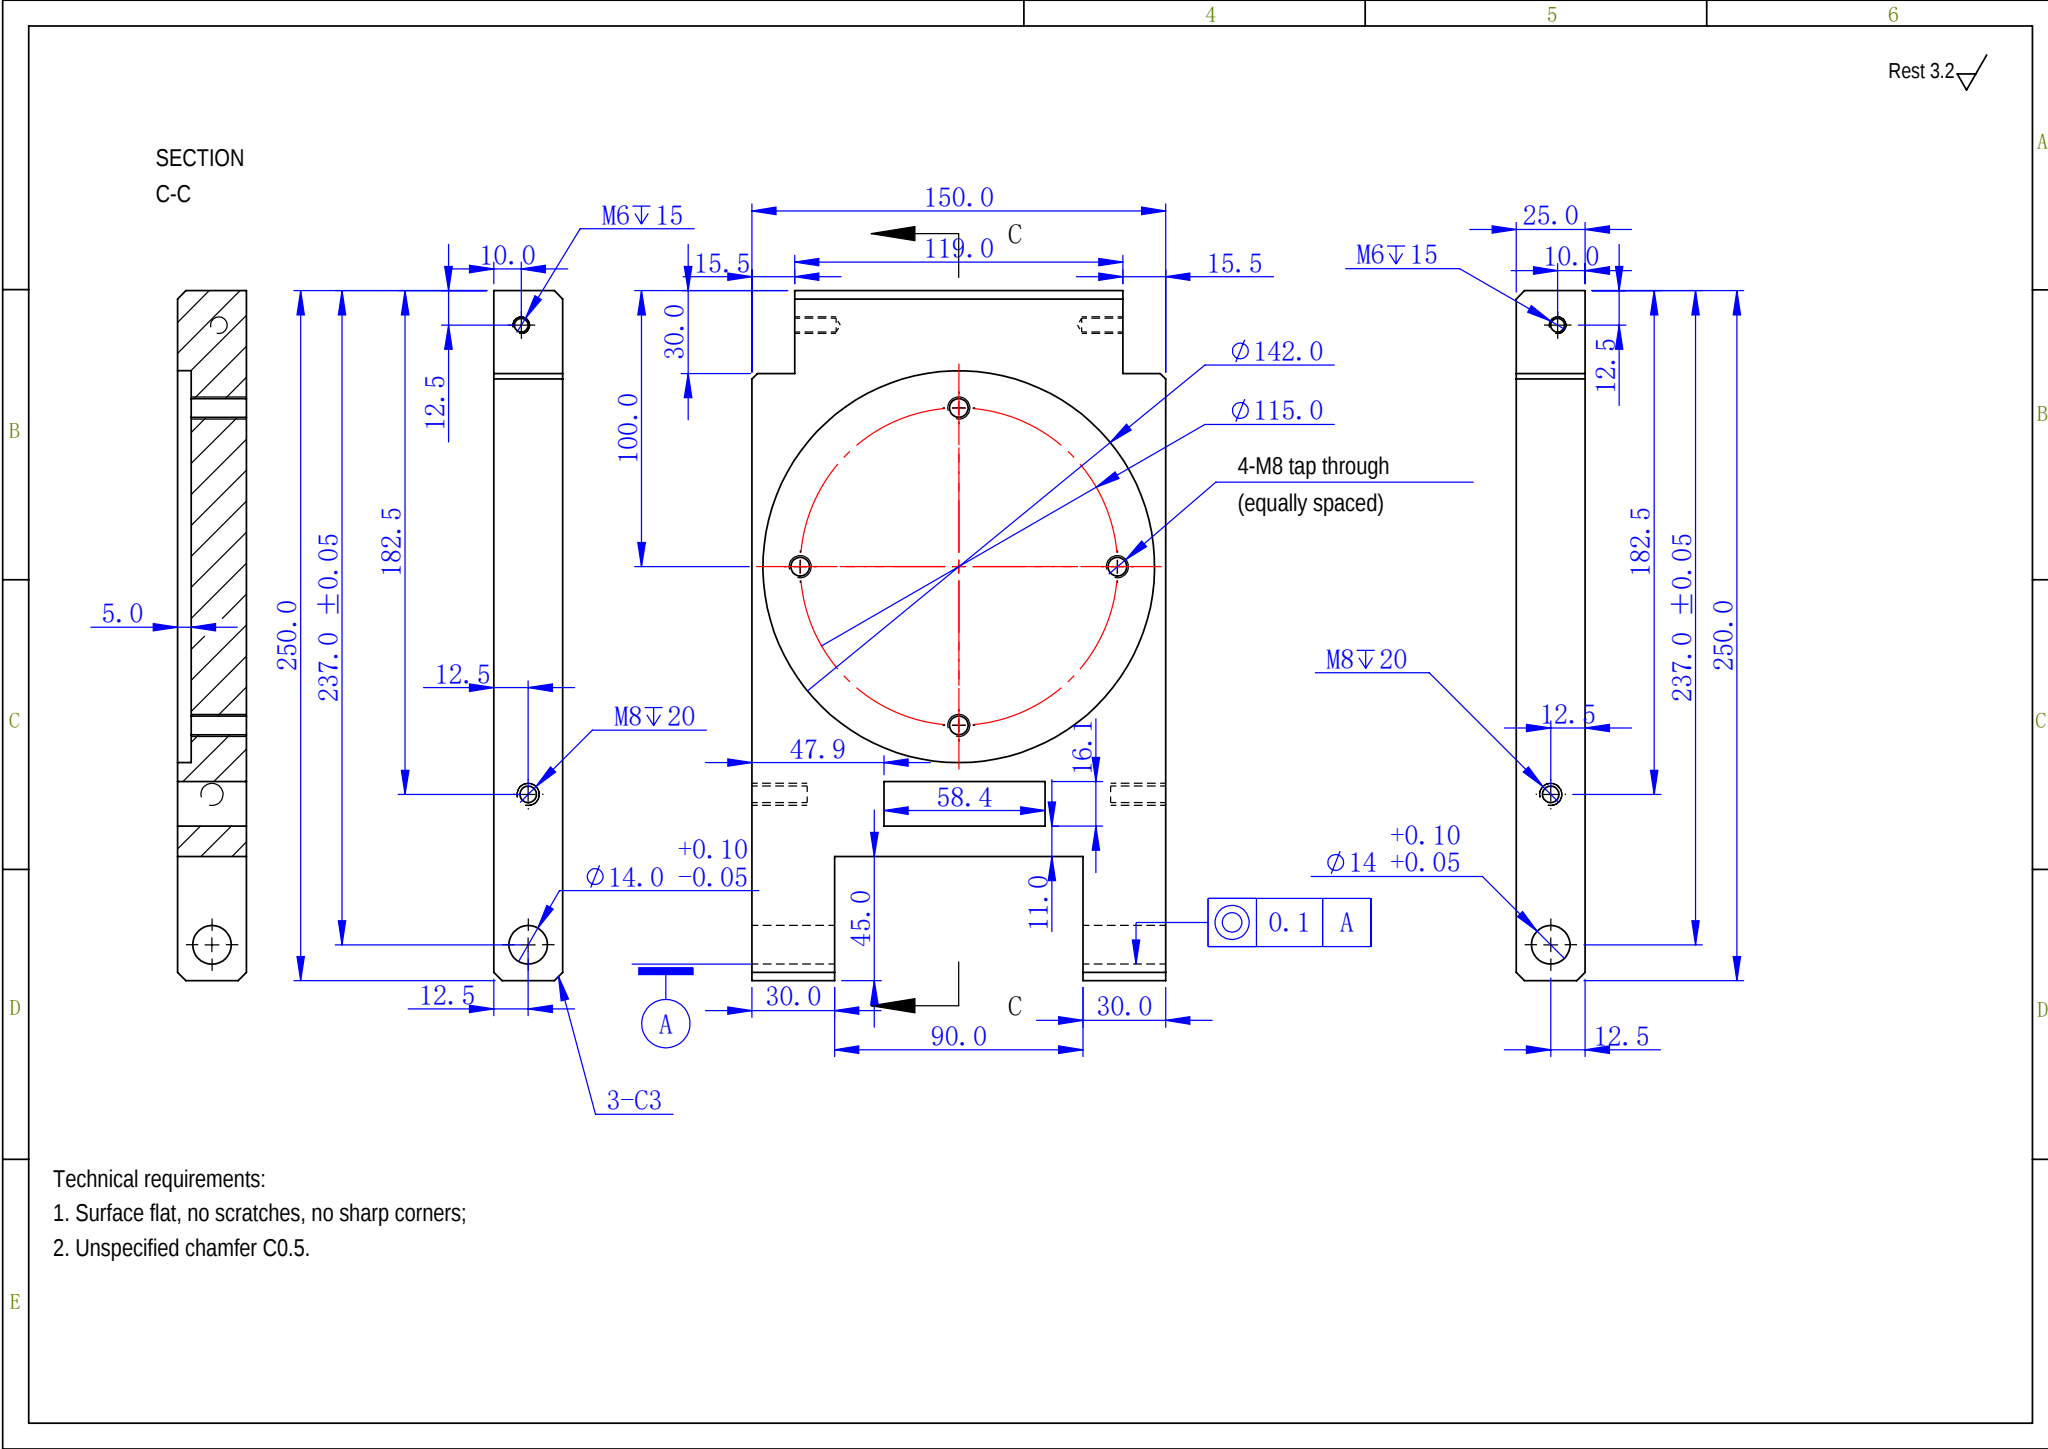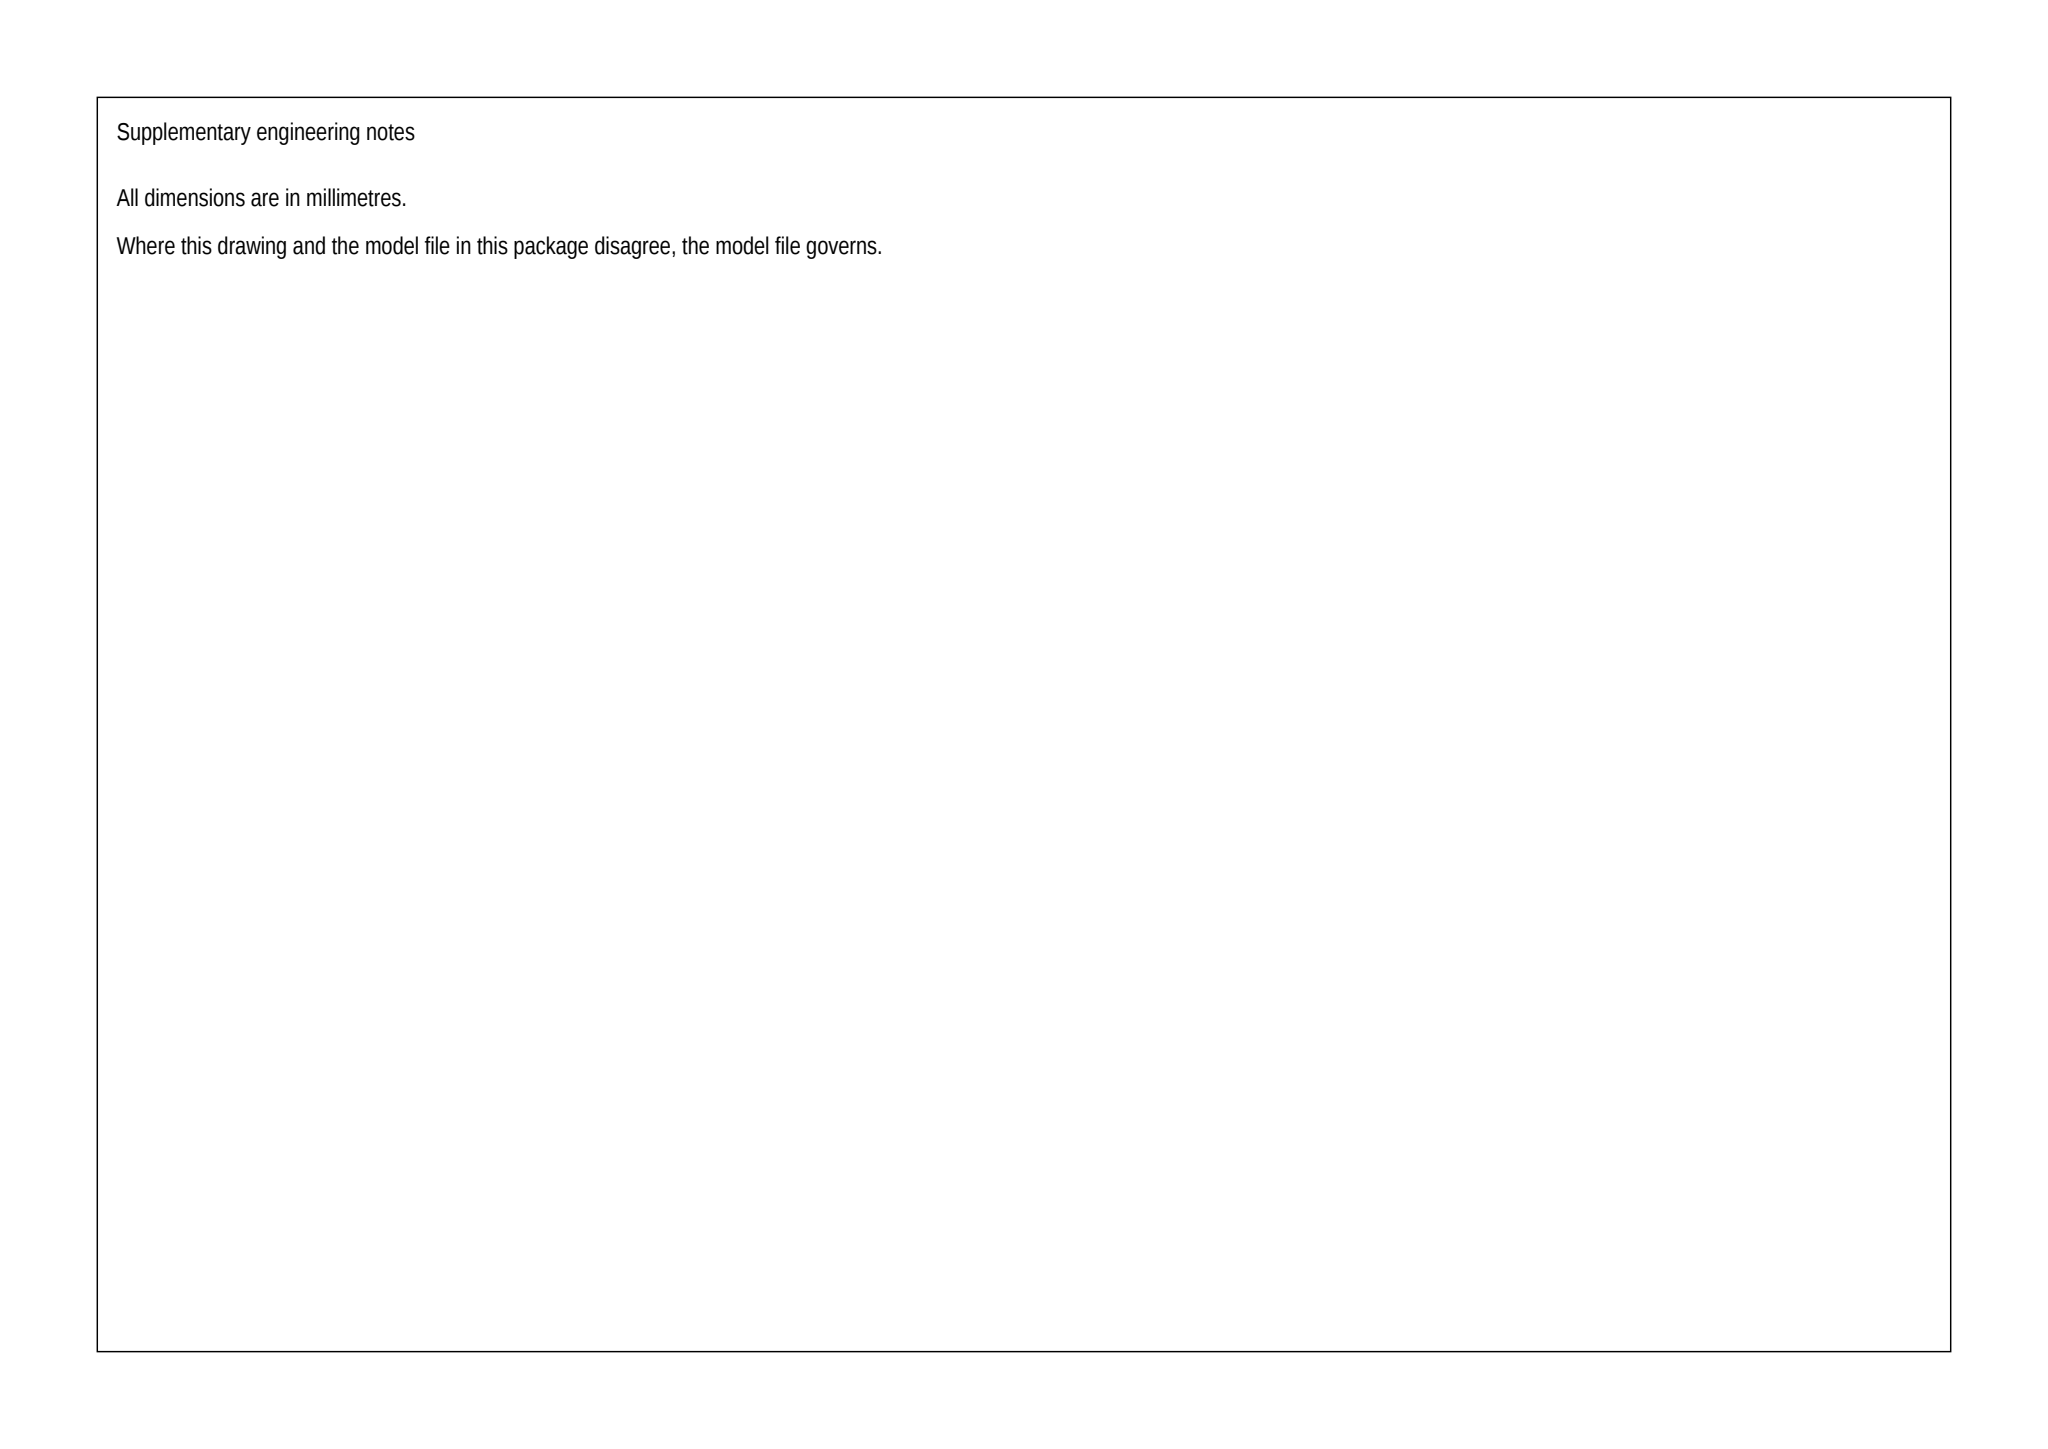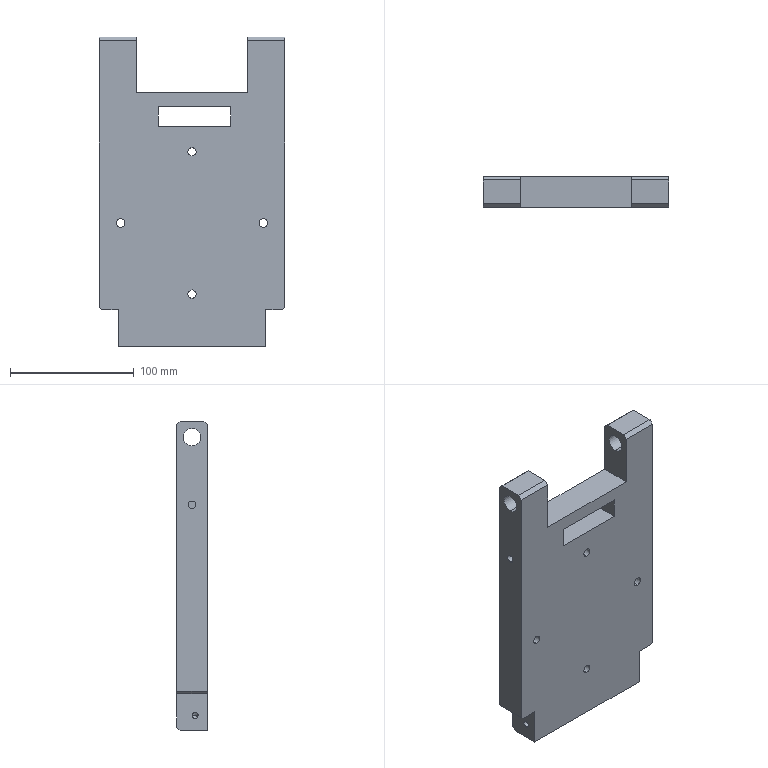Part | SolidWorks | mm | 1 solid | 54 faces | box 150 x 25 x 250 mm | volume 695225 mm3 | plane 28 | cylinder 22 | cone 4 | commonest cylinder face diameters 6.8 x8 14 x4 6 x4 5 x4 142 x2